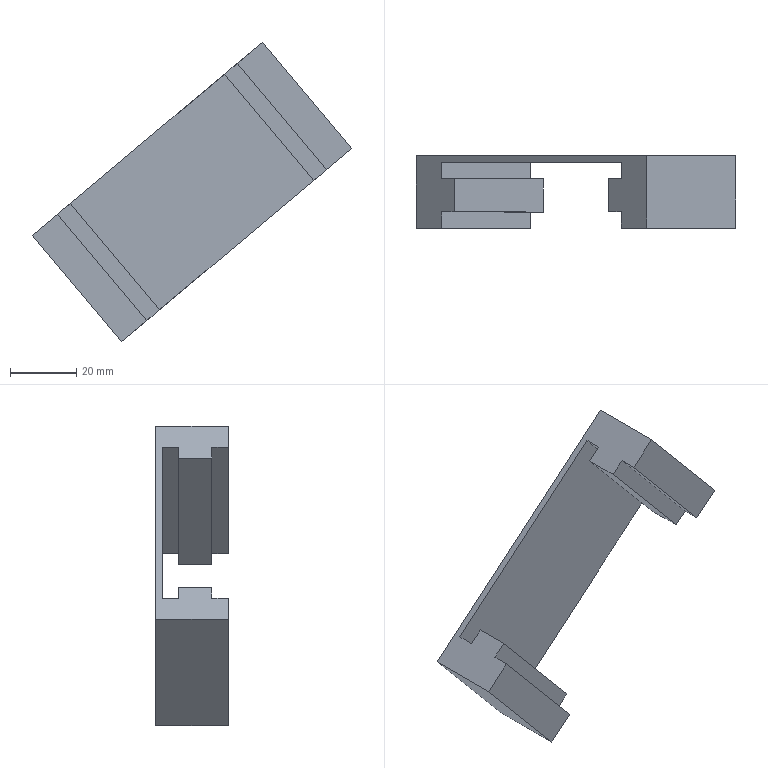Component | NX | MODEL5 | 1 solid | 18 faces | volume 28644 mm3 | plane 18